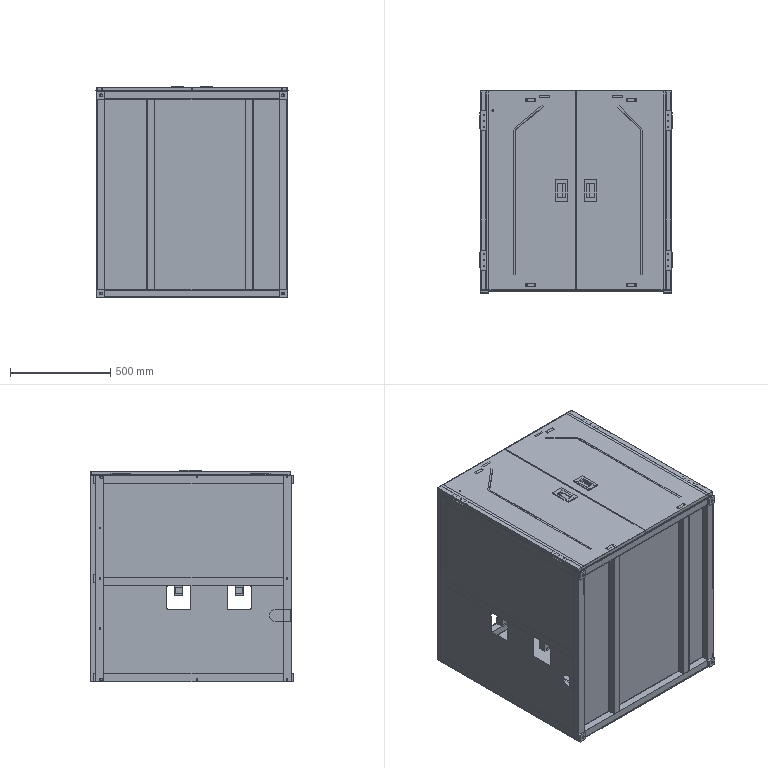Assembly | SolidWorks | mm | 26 component files | 83 solids | 1460 faces | box 959.2 x 1010 x 1056.7 mm | volume 15689456 mm3 | plane 913 | cylinder 531 | torus 16 | commonest cylinder face diameters 4.2 x68 6 x54 4 x52 5 x48 6.5 x48 8.5 x44 3 x30 14 x28
Bill of materials:
SYM0545-81-107 | 2 | PP Copolymer | Thick rectangular block (nearly square in face view) with two round through-holes in a line near one edge.
SYM0590-81-102 | 1 | Plain Carbon Steel | Thin flat rectangular plate, long and narrow, with no visible holes or cutouts.
SYM0590-81-103 | 1 | Plain Carbon Steel | Thin flat rectangular plate, wider in proportion than part-1 (about 2:1 height to width), with no visible features.
SYM0590-81-104 | 1 | Plain Carbon Steel | Thin flat rectangular strip or plate, very narrow and elongated, with no visible holes.
SYM0636-81-109 | 4 | AISI 304 | Cube-shaped thin-walled open box: four side walls and a closed bottom, with the top open. One face, apparently the bottom, has a single central round hole.
SYM0671-81-101 | 1 | AISI 304 | Open rectilinear frame built from square or rectangular section bars: corner uprights, intermediate uprights, top and bottom perimeter rails, intermediate horizontal rails, a smaller sub-frame near the bottom, diagonal corner braces in one elevation, and short stub tabs on some members. Part of the top perimeter is missing, so the frame is open on that side.
SYM0671-81-108 | 1 | AISI 304 | Rectangular flat bar with four small round through-holes: two near each end, aligned along a line parallel to the long edge and offset toward one long edge.
SYM0671-81-104 | 1 |  | Thin square sheet panel with two square cutouts with rounded corners side by side in the lower middle area, plus small holes around the perimeter, including some keyhole-like shapes at the corners.
SYM0671-81-105 | 1 |  | Thin square sheet panel similar to part-01931d67, with two square cutouts with rounded corners and perimeter holes, plus an edge slot with a rounded end, open to one side edge below the cutouts.
SYM0671-81-106 | 1 | Plain Carbon Steel | Thin square sheet panel with no large cutouts and a series of small holes near the edges, including keyhole-shaped holes at two adjacent corners.
SYM0671-81-201 | 1 | Steel | Flat rectangular plate (about 2:1) of moderate thickness, with one small rectangular cutout near one long edge surrounded by four small holes, and a single small round hole near an opposite corner.
SYM0671-81-202 | 1 | AISI 304 | Long angle-section (L-profile) member with small holes spaced along its length. It has one long straight segment and a short segment joined to it at an angle, giving a bent or mitered shape in one view.
SYMA1-51a_mis_shhpsk6-3 | 4 |  | Elongated U-shaped part: two parallel flat rectangular leaves joined along one long edge by a rounded cylindrical end section, with three evenly spaced round holes along the leaves.
SYMA1-51a_mis_uwuan109.5-b | 2 |  | Thin rectangular plate with a rectangular slot-shaped recess or opening in its upper face. A rectangular block and small cylindrical pins stick out from the underside.
SYMA1-51-omr_gls-s1 | 2 | ﾃﾞﾙﾘﾝ | Elongated block-shaped part with a flat top flange. The flange has rounded ends, each with a round hole, and sits over a narrower stepped rectangular body that has notches, a rib and part-cylindrical features on one side.
SYM0671-81-301 | 1 | Steel | Large thin flat rectangular panel with one small rectangular through cutout near one long edge, surrounded by four small holes. The underside edge appears to have shallow notches or steps.
SYM0671-81-302 | 1 | AISI 304 | Long, very thin, narrow strip of sheet-like material bent near one end into a short angled leg, with small holes along its length.
Mates:
1. concentric | assembly face at (-392.749, -496.857, 10.518) dir (0, 0, -1) r 2 | SYM0671-81-106-2 face at (-392.749, -496.857, -0.6824) dir (0, 0, 1) r 3
2. concentric | assembly face at (72.251, -496.857, 10.518) dir (0, 0, -1) r 2 | SYM0671-81-106-2 face at (72.251, -496.857, -0.6824) dir (0, 0, 1) r 3
3. coincident | assembly face at (-399.749, -516.857, 0.5176) dir (0, 0, -1) | SYM0671-81-106-2 face at (-402.749, 483.143, 0.5176) dir (0, 0, 1)
4. coincident | assembly face at (-127.749, 455.143, 993.518) dir (1, 0, 0) | SYM0545-81-107-1 face at (-127.749, 433.143, 1030.518) dir (-1, 0, 0)
5. coincident | assembly face at (-167.749, 468.143, 1030.518) dir (0, 1, 0) | SYM0545-81-107-1 face at (-117.749, 468.143, 1030.518) dir (0, 1, 0)
6. coincident | assembly face at (563.82, 455.143, 1030.518) dir (0, 0, 1) | SYM0545-81-107-1 face at (-117.749, 468.143, 1030.518) dir (0, 0, 1)
7. coincident | assembly face at (322.251, 455.143, 993.518) dir (-1, 0, 0) | SYM0545-81-107-2 face at (322.251, 433.143, 990.518) dir (1, 0, 0)
8. coincident | assembly face at (563.82, 455.143, 1030.518) dir (0, 0, 1) | SYM0545-81-107-2 face at (312.251, 468.143, 1030.518) dir (0, 0, 1)
9. coincident | assembly face at (362.251, 468.143, 990.518) dir (0, 1, 0) | SYM0545-81-107-2 face at (312.251, 468.143, 990.518) dir (0, 1, 0)
10. distance | assembly face at (-362.749, 468.143, 990.518) dir (0, 1, 0) | SYM0671-81-200-1/SYM0671-81-201-1 face at (-402.749, 483.143, 1031.018) dir (0, 1, 0)
11. coincident | assembly face at (-399.749, -516.857, 1030.518) dir (0, 0, 1) | SYM0671-81-200-1/SYMA1-51a_mis_shhpsk6-3-1 face at (-402.749, 372.143, 1030.518) dir (0, 0, -1)
12. coincident | SYM0671-81-200-1/SYM0671-81-201-1 face at (-402.749, 483.143, 1051.018) dir (0, 0, 1) | SYM0671-81-300-1/SYM0671-81-301-1 face at (73.251, -512.857, 1051.018) dir (0, 0, 1)
13. coincident | SYM0671-81-200-1/SYM0671-81-201-1 face at (-402.749, 483.143, 1031.018) dir (0, 1, 0) | SYM0671-81-300-1/SYM0671-81-301-1 face at (73.251, 483.143, 1031.018) dir (0, 1, 0)
14. concentric | assembly face at (-392.749, -496.857, 1020.518) dir (-1, 0, 0) r 2 | SYM0671-81-105-2 face at (-403.949, -496.857, 1020.518) dir (1, 0, 0) r 3
15. coincident | assembly face at (-402.749, -516.857, 993.518) dir (-1, 0, 0) | SYM0671-81-105-2 face at (-402.749, 473.143, 1030.518) dir (1, 0, 0)
16. concentric | assembly face at (537.251, -496.857, 1020.518) dir (1, 0, 0) r 2 | SYM0671-81-104-2 face at (548.451, -496.857, 1020.518) dir (-1, 0, 0) r 3
17. coincident | assembly face at (547.251, -516.857, 993.518) dir (1, 0, 0) | SYM0671-81-104-2 face at (547.251, 483.143, 1030.518) dir (-1, 0, 0)
18. coincident | SYM0671-81-104-2 face at (547.251, 483.143, 1030.518) dir (-1, 0, 0) | SYM0671-81-300-1/SYM0671-81-301-1 face at (547.251, 483.143, 1031.018) dir (1, 0, 0)
19. concentric | assembly face at (537.251, -46.857, 1020.518) dir (1, 0, 0) r 2 | SYM0671-81-104-2 face at (548.451, -46.857, 1020.518) dir (-1, 0, 0) r 3
20. concentric | assembly face at (-392.749, -496.857, 10.518) dir (-1, 0, 0) r 2 | SYM0671-81-105-2 face at (-403.949, -496.857, 10.518) dir (1, 0, 0) r 3
21. coincident | SYM0671-81-101-2 face at (-326.284, -935, 20) dir (0, 1, 0) | SYM0590-81-103-1 face at (-286.284, -935, 990) dir (0, 1, 0)
22. coincident | SYM0671-81-101-2 face at (-286.284, -975, 20) dir (1, 0, 0) | SYM0590-81-103-1 face at (-286.284, -935, 40) dir (-1, 0, 0)
23. coincident | SYM0671-81-101-2 face at (-556.284, -975, 990) dir (0, 0, -1) | SYM0590-81-103-1 face at (-286.284, -935, 990) dir (0, 0, 1)
24. coincident | SYM0671-81-101-2 face at (-326.284, -935, 20) dir (0, 1, 0) | SYM0590-81-102-3 face at (-536.284, -935, 990) dir (0, 1, 0)
25. coincident | SYM0671-81-101-2 face at (-556.284, -975, 990) dir (0, 0, -1) | SYM0590-81-102-3 face at (-536.284, -935, 990) dir (0, 0, 1)
26. coincident | SYM0671-81-101-2 face at (-536.284, -975, 20) dir (1, 0, 0) | SYM0590-81-102-3 face at (-536.284, -935, 40) dir (-1, 0, 0)
27. coincident | SYM0671-81-101-2 face at (-556.284, -935, 1030) dir (0, 1, 0) | SYM0590-81-104-2 face at (203.716, -935, 990) dir (0, 1, 0)
28. coincident | SYM0671-81-101-2 face at (203.716, -975, 20) dir (1, 0, 0) | SYM0590-81-104-2 face at (203.716, -935, 40) dir (-1, 0, 0)
29. coincident | SYM0671-81-101-2 face at (-556.284, -975, 990) dir (0, 0, -1) | SYM0590-81-104-2 face at (203.716, -935, 990) dir (0, 0, 1)
30. coincident | SYM0671-81-101-2 face at (-306.284, -656, 260) dir (0, 1, 0) | SYM0671-81-108-1 face at (-206.784, -656, 260) dir (0, -1, 0)
31. coincident | SYM0671-81-101-2 face at (-536.284, -435, 469) dir (0, 0, -1) | SYM0636-81-109-1 face at (-536.284, -395, 469) dir (0, 0, 1)
32. coincident | SYM0671-81-101-2 face at (-536.284, -395, 469) dir (0, 1, 0) | SYM0636-81-109-1 face at (-576.284, -395, 469) dir (0, 1, 0)
33. coincident | SYM0671-81-101-2 face at (-576.284, -395, 469) dir (-1, 0, 0) | SYM0636-81-109-1 face at (-576.284, -395, 469) dir (-1, 0, 0)
34. coincident | SYM0671-81-101-2 face at (-306.284, -656, 300) dir (0, 0, 1) | SYM0671-81-108-1 face at (-16.784, -656, 300) dir (0, 0, 1)
35. distance | SYM0671-81-108-1 face at (-206.784, -656, 300) dir (-1, 0, 0) | SYM0671-81-101-2 face at (-326.284, -656, 280) dir (-1, 0, 0)
36. coincident | SYM0671-81-201-1 face at (0, 996, 0) dir (0, 0, 1) | SYMA1-51a_mis_uwuan109.5-b-1 face at (435, 552.75, 0) dir (0, 0, -1)
37. concentric | SYM0671-81-201-1 face at (384, 454, 0.001) dir (0, 0, -1) r 2.5 | SYMA1-51a_mis_uwuan109.5-b-1 face at (384, 454, -9) dir (0, 0, 1) r 2
38. concentric | SYM0671-81-201-1 face at (422, 542, 0.001) dir (0, 0, -1) r 2.5 | SYMA1-51a_mis_uwuan109.5-b-1 face at (422, 542, -9) dir (0, 0, 1) r 2
39. concentric | SYM0671-81-201-1 face at (16, 876, -1.5) dir (0, 0, -1) r 2 | SYMA1-51a_mis_shhpsk6-3-1 face at (16, 876, -11.3) dir (0, 0, -1) r 3.25
40. concentric | SYM0671-81-201-1 face at (16, 816, -1.5) dir (0, 0, -1) r 2 | SYMA1-51a_mis_shhpsk6-3-1 face at (16, 816, -11.3) dir (0, 0, -1) r 3.25
41. coincident | SYM0671-81-201-1 face at (1.5, 896, -11.3) dir (0, 0, -1) | SYMA1-51a_mis_shhpsk6-3-1 face at (0, 885, -11.3) dir (0, 0, 1)
42. concentric | SYM0671-81-201-1 face at (296, 967, -10.5) dir (0, 0, -1) r 1.5 | SYMA1-51-omr_gls-s1-1 face at (296, 967, -16.5) dir (0, 0, -1) r 1.9
43. concentric | SYM0671-81-201-1 face at (336, 967, -10.5) dir (0, 0, -1) r 1.5 | SYMA1-51-omr_gls-s1-1 face at (336, 967, -16.5) dir (0, 0, -1) r 1.9
44. coincident | SYM0671-81-201-1 face at (341, 962, -16.5) dir (0, 0, -1) | SYMA1-51-omr_gls-s1-1 face at (341, 962, -16.5) dir (0, 0, 1)
45. coincident | SYM0671-81-201-1 face at (0, 996, -1.5) dir (0, 0, -1) | SYM0671-81-202-1 face at (311.388, 915.702, -1.5) dir (0, 0, 1)
46. distance | SYM0671-81-202-1 face at (174, 800, -12) dir (1, 0, 0) | SYM0671-81-201-1 face at (474, 996, -20) dir (1, 0, 0)
47. distance | SYM0671-81-202-1 face at (173.5, 80, -12) dir (0, -1, 0) | SYM0671-81-201-1 face at (0, 0, -20) dir (0, -1, 0)
48. coincident | SYM0671-81-301-1 face at (-474, 0, 0) dir (0, 0, 1) | SYMA1-51a_mis_uwuan109.5-b-1 face at (-435, 443.25, 0) dir (0, 0, -1)
49. concentric | SYM0671-81-301-1 face at (-422, 542, 0.001) dir (0, 0, -1) r 2.5 | SYMA1-51a_mis_uwuan109.5-b-1 face at (-422, 542, -9) dir (0, 0, 1) r 2
50. concentric | SYM0671-81-301-1 face at (-384, 454, 0.001) dir (0, 0, -1) r 2.5 | SYMA1-51a_mis_uwuan109.5-b-1 face at (-384, 454, -9) dir (0, 0, 1) r 2
51. coincident | SYM0671-81-301-1 face at (-1.5, 896, -11.3) dir (0, 0, -1) | SYMA1-51a_mis_shhpsk6-3-1 face at (0, 885, -11.3) dir (0, 0, 1)
52. concentric | SYM0671-81-301-1 face at (-286, 967, -10.5) dir (0, 0, -1) r 1.5 | SYMA1-51-omr_gls-s1-1 face at (-286, 967, -16.5) dir (0, 0, -1) r 1.9
53. concentric | SYM0671-81-301-1 face at (-246, 967, -10.5) dir (0, 0, -1) r 1.5 | SYMA1-51-omr_gls-s1-1 face at (-246, 967, -16.5) dir (0, 0, -1) r 1.9
54. coincident | SYM0671-81-301-1 face at (-241, 962, -16.5) dir (0, 0, -1) | SYMA1-51-omr_gls-s1-1 face at (-241, 962, -16.5) dir (0, 0, 1)
55. concentric | SYM0671-81-301-1 face at (-16, 816, 0) dir (0, 0, -1) r 2 | SYMA1-51a_mis_shhpsk6-3-1 face at (-16, 816, -20.5) dir (0, 0, 1) r 3.25
56. concentric | SYM0671-81-301-1 face at (-16, 876, 0) dir (0, 0, -1) r 2 | SYMA1-51a_mis_shhpsk6-3-1 face at (-16, 876, -20.5) dir (0, 0, 1) r 3.25
57. coincident | SYM0671-81-301-1 face at (-474, 0, -1.5) dir (0, 0, -1) | SYM0671-81-302-1 face at (-153.5, 80, -1.5) dir (0, 0, 1)
58. distance | SYM0671-81-302-1 face at (-153.5, 80, -1.5) dir (0, -1, 0) | SYM0671-81-301-1 face at (-474, 0, -20) dir (0, -1, 0)
59. distance | SYM0671-81-302-1 face at (-154, 800, -12) dir (-1, 0, 0) | SYM0671-81-301-1 face at (-474, 996, -20) dir (-1, 0, 0)